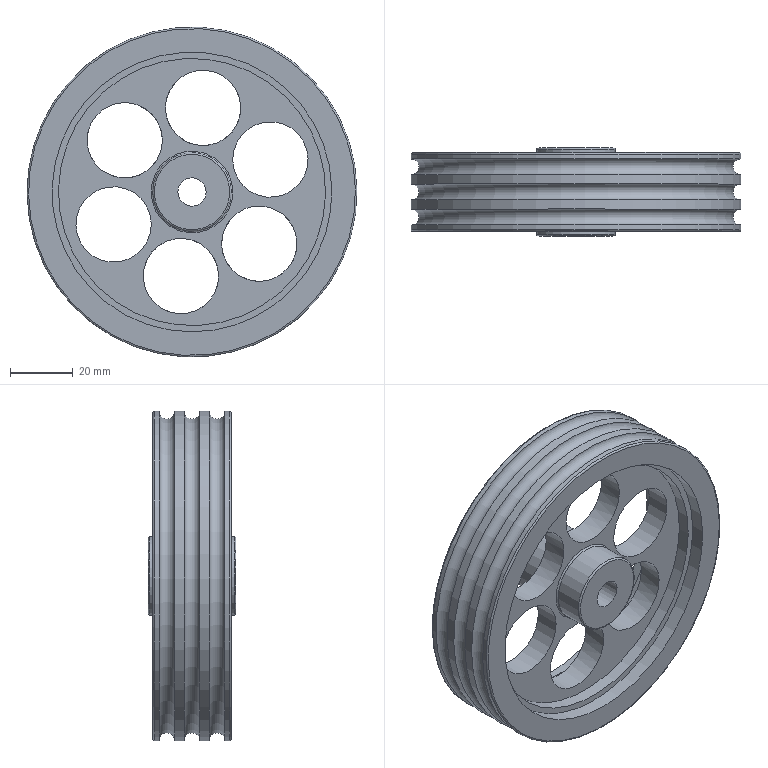Component | NX | PULLEY_2 | 1 solid | 34 faces | volume 91856 mm3 | cylinder 17 | torus 9 | plane 8 | commonest cylinder face diameters 24 x6 105 x4 89 x2 85 x2 25 x2 9 x1